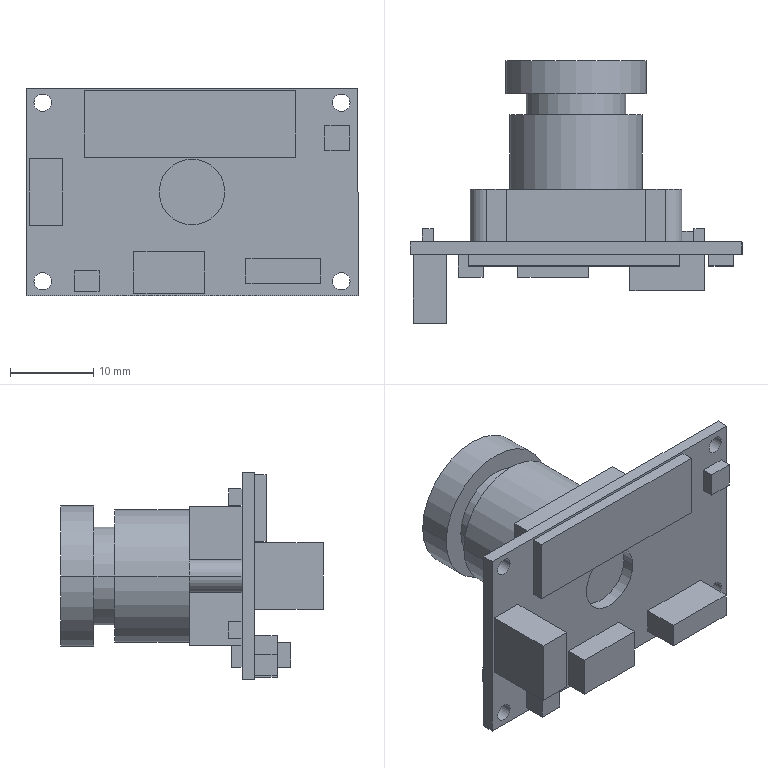Component | SolidWorks | Actuator-1 | 1 solid | 85 faces | box 40 x 31.65 x 25 mm | volume 7243 mm3 | plane 66 | cylinder 19 | commonest cylinder face diameters 2.1 x8 4 x3 16 x2 12 x2 17 x2 7.908 x2
build123d program:
from build123d import *

# Parameters (mm, degrees)
SKETCH1_W           = 40
SKETCH1_H           = 25
SKETCH1_R           = 3.954
SKETCH1_R_2         = 1.05
BOSS_EXTRUDE1_DEPTH = 1.5
SKETCH3_W           = 25.5
SKETCH3_H           = 8
SKETCH3_W_2         = 3
SKETCH3_H_2         = 3
BOSS_EXTRUDE2_DEPTH = 1.4
SKETCH4_W           = 3
SKETCH4_H           = 2.5
SKETCH4_W_2         = 8.5
SKETCH4_H_2         = 5
BOSS_EXTRUDE3_DEPTH = 2.74
SKETCH5_W           = 4
SKETCH5_H           = 8
BOSS_EXTRUDE4_DEPTH = 8.3
SKETCH6_W           = 9
SKETCH6_H           = 3
BOSS_EXTRUDE5_DEPTH = 4.35
SKETCH7_W           = 1.3
SKETCH7_H           = 2
BOSS_EXTRUDE6_DEPTH = 1.6
SKETCH8_W           = 3
SKETCH8_H           = 5
BOSS_EXTRUDE7_DEPTH = 1.3
SKETCH9_W           = 16.8
SKETCH9_H           = 16.8
BOSS_EXTRUDE8_DEPTH = 6.35
BOSS_EXTRUDE9_DEPTH = 6.35


with BuildPart() as part:
    # Sketch1 → Boss-Extrude1 (new body)
    with BuildSketch(Plane.XY):
        Rectangle(SKETCH1_W, SKETCH1_H)
        Circle(SKETCH1_R, mode=Mode.SUBTRACT)
        with Locations((-18, 10.75)):
            Circle(SKETCH1_R_2, mode=Mode.SUBTRACT)
        with Locations((18, 10.75)):
            Circle(SKETCH1_R_2, mode=Mode.SUBTRACT)
        with Locations((18, -10.75)):
            Circle(SKETCH1_R_2, mode=Mode.SUBTRACT)
        with Locations((-18, -10.75)):
            Circle(SKETCH1_R_2, mode=Mode.SUBTRACT)
    extrude(amount=BOSS_EXTRUDE1_DEPTH)

    # Sketch3 → Boss-Extrude2 (add)
    with BuildSketch(Plane.XY.offset(1.5)):
        with Locations((-0.25, 8.2)):
            Rectangle(SKETCH3_W, SKETCH3_H)
        with Locations((17.5, 6.5)):
            Rectangle(SKETCH3_W_2, SKETCH3_H_2)
    extrude(amount=BOSS_EXTRUDE2_DEPTH)

    # Sketch4 → Boss-Extrude3 (add)
    with BuildSketch(Plane.XY.offset(1.5)):
        with Locations((-12.7, -10.75)):
            Rectangle(SKETCH4_W, SKETCH4_H)
        with Locations((-2.75, -9.7)):
            Rectangle(SKETCH4_W_2, SKETCH4_H_2)
    extrude(amount=BOSS_EXTRUDE3_DEPTH)

    # Sketch5 → Boss-Extrude4 (add)
    with BuildSketch(Plane.XY.offset(1.5)):
        with Locations((-17.62, 0)):
            Rectangle(SKETCH5_W, SKETCH5_H)
    extrude(amount=BOSS_EXTRUDE4_DEPTH)

    # Sketch6 → Boss-Extrude5 (add)
    with BuildSketch(Plane.XY.offset(1.5)):
        with Locations((11, -9.5)):
            Rectangle(SKETCH6_W, SKETCH6_H)
    extrude(amount=BOSS_EXTRUDE5_DEPTH)

    # Sketch7 → Boss-Extrude6 (add)
    with BuildSketch(Plane(origin=(0, 0, 0), x_dir=(-1, 0, 0), z_dir=(0, 0, -1))):
        with Locations((-14.85, 9.5)):
            Rectangle(SKETCH7_W, SKETCH7_H)
        with Locations((17.85, -6.5)):
            Rectangle(SKETCH7_W, SKETCH7_H)
    extrude(amount=BOSS_EXTRUDE6_DEPTH)

    # Sketch8 → Boss-Extrude7 (add)
    with BuildSketch(Plane(origin=(0, 0, 0), x_dir=(-1, 0, 0), z_dir=(0, 0, -1))):
        with Locations((-13, -8.5)):
            Rectangle(SKETCH8_W, SKETCH8_H)
    extrude(amount=BOSS_EXTRUDE7_DEPTH)

    # Sketch9 → Boss-Extrude8 (add)
    with BuildSketch(Plane(origin=(0, 0, 0), x_dir=(-1, 0, 0), z_dir=(0, 0, -1))):
        Rectangle(SKETCH9_W, SKETCH9_H)
    extrude(amount=BOSS_EXTRUDE8_DEPTH)

    # Sketch10 → Boss-Extrude9 (add)
    with BuildSketch(Plane(origin=(0, 0, -6.35), x_dir=(-1, 0, 0), z_dir=(0, 0, -1))):
        with BuildLine():
            Line((-10.75, 2), (10.75, 2))
            ThreePointArc((10.75, 2), (12.75, 0), (10.75, -2))
            Line((10.75, -2), (-10.75, -2))
            ThreePointArc((-10.75, -2), (-12.75, 0), (-10.75, 2))
        make_face()
    extrude(amount=-BOSS_EXTRUDE9_DEPTH)

    # Sketch11 → Revolve1 (revolve)
    with BuildSketch(Plane(origin=(0, 0, 0), x_dir=(1, 0, 0), z_dir=(0, 1, 0)), mode=Mode.PRIVATE) as revolve1_sk:
        Polygon((0, 21.85), (-8.5, 21.85), (-8.5, 17.85), (-6, 17.85), (-6, 15.35), (-8, 15.35), (-8, 6.35), (0, 6.35), align=None)
    revolve(revolve1_sk.sketch.rotate(Axis((0, 0, 0), (0, 0, -1)), 180), axis=Axis((0, 0, 0), (0, 0, -1)))


solid = part.part

# Placed as in the assembly
solid = solid.moved(Location((-50.116, 108.825, 1018.85), (90, 0, 0)))